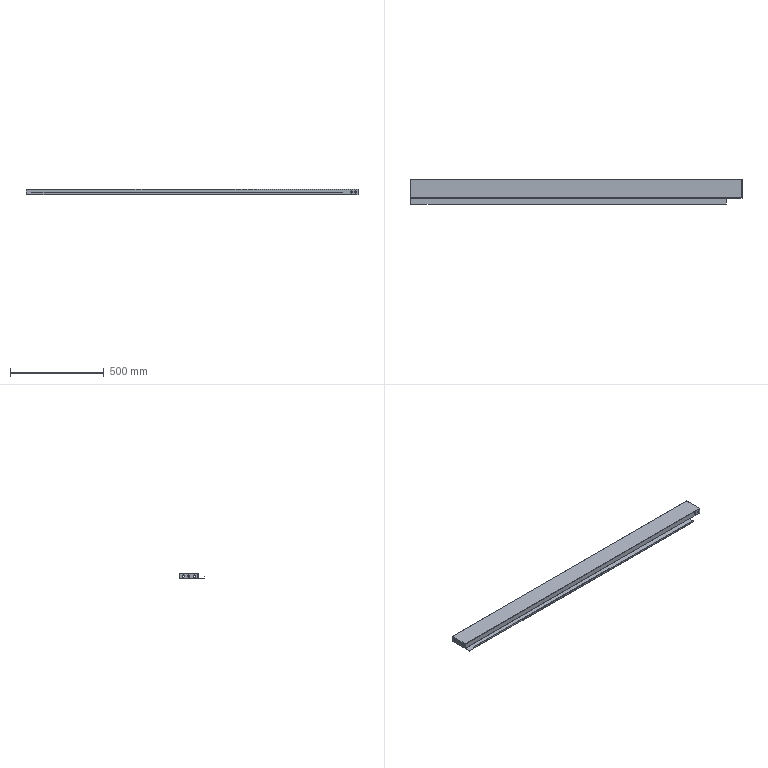Component | SolidWorks | UpperCrossbeam-1 | 1 solid | 108 faces | volume 524881 mm3 | plane 62 | cylinder 46 | commonest cylinder face diameters 11 x34 3.4 x6 0.4 x6